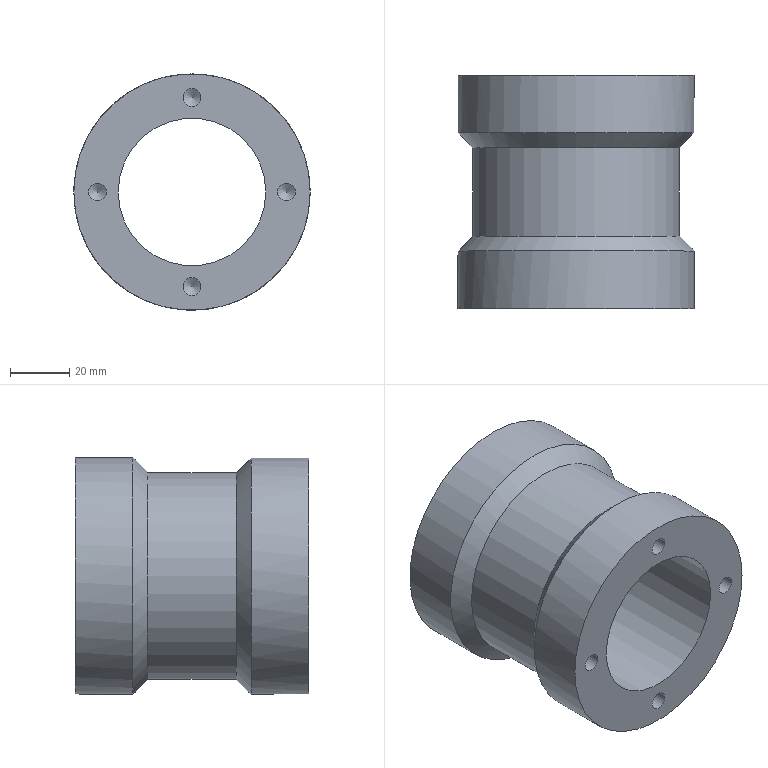Component | NX | CYLINDER_BARREL | 1 solid | 24 faces | volume 197767 mm3 | cylinder 12 | cone 10 | plane 2 | commonest cylinder face diameters 6 x8 80 x2 50 x1 70 x1